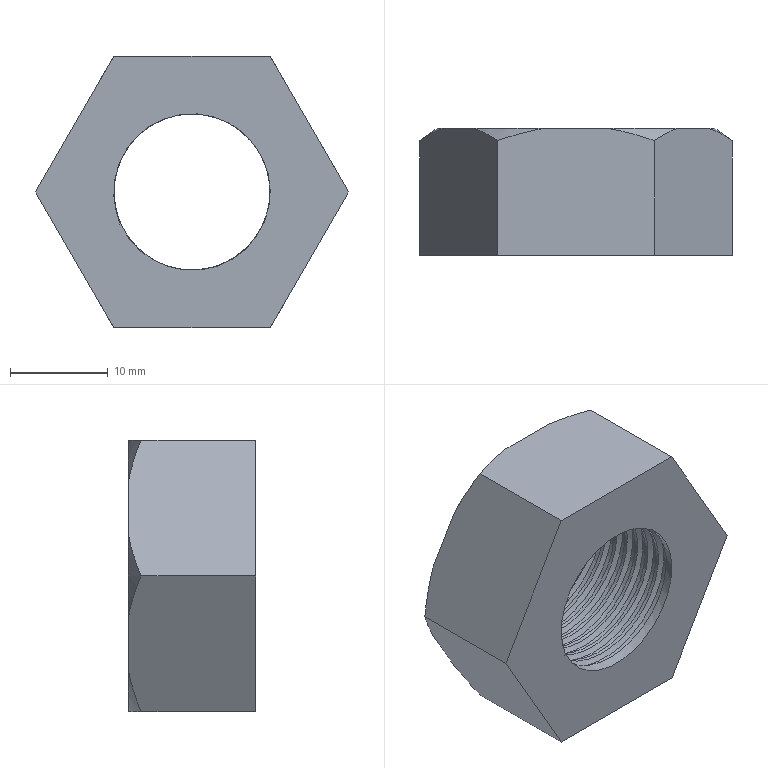Component | NX | NUT_M16 | 1 solid | 19 faces | volume 5831 mm3 | plane 9 | cone 6 | cylinder 2 | spline 2 | commonest cylinder face diameters 16 x1 17 x1